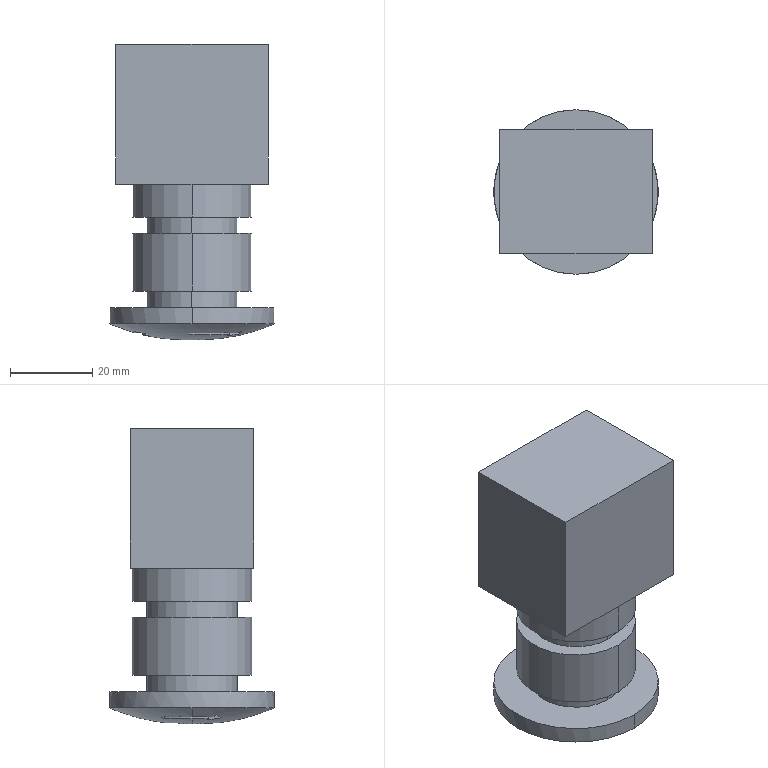Component | SolidWorks | EmergencyStopButton-0-1 | 1 solid | 46 faces | volume 62839 mm3 | plane 28 | cylinder 16 | spline 2 | commonest cylinder face diameters 29 x4 22 x4 24 x3 28 x3 40 x2